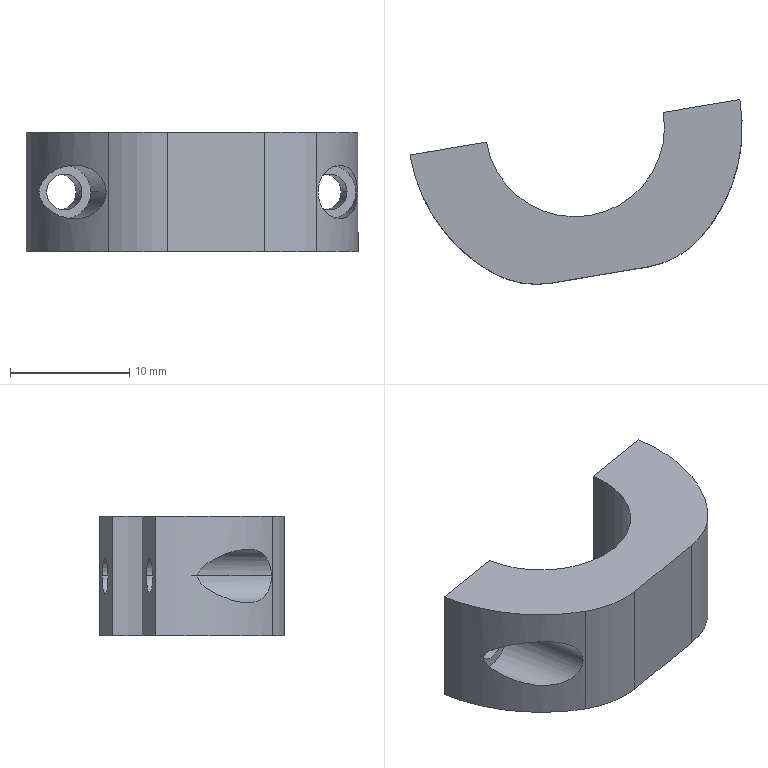Component | SolidWorks | ConnectingRod1-1-1 | 1 solid | 21 faces | box 27.81 x 15.47 x 10 mm | volume 1858 mm3 | cylinder 14 | plane 7 | commonest cylinder face diameters 4.5 x4 3 x4 15 x4 28 x2
build123d program:
from build123d import *

# Parameters (mm, degrees)
BOSS_EXTRUDE1_DEPTH = 20
SKETCH2_R           = 6
CUT_EXTRUDE1_DEPTH  = 12
SKETCH3_R           = 9
CUT_EXTRUDE2_DEPTH  = 74.973
SKETCH4_W           = 60.236
SKETCH4_H           = 18.31
CUT_EXTRUDE3_DEPTH  = 89.724
FILLET1_R           = 30
SCALE1_SCALE        = 0.25


with BuildPart() as part:
    # Sketch1 → Boss-Extrude1 (new, symmetric)
    with BuildSketch(Plane(origin=(0, 0, 0), x_dir=(1, 0, 0), z_dir=(0, 1, 0))):
        with BuildLine():
            Line((-56, 0), (-30, 0))
            ThreePointArc((-30, 0), (0, 30), (30, 0))
            Line((30, 0), (56, 0))
            ThreePointArc((56, 0), (0, 56), (-56, 0))
        make_face()
    extrude(amount=BOSS_EXTRUDE1_DEPTH, both=True)

    # Sketch2 → Cut-Extrude1 (cut)
    with BuildSketch(Plane.XY):
        with Locations((-45, 0)):
            Circle(SKETCH2_R)
        with Locations((45, 0)):
            Circle(SKETCH2_R)
    extrude(amount=-CUT_EXTRUDE1_DEPTH, mode=Mode.SUBTRACT)

    # Sketch3 → Cut-Extrude2 (cut, through all)
    with BuildSketch(Plane.XY.offset(-12)):
        with Locations((-45, 0)):
            Circle(SKETCH3_R)
        with Locations((45, 0)):
            Circle(SKETCH3_R)
    extrude(amount=-CUT_EXTRUDE2_DEPTH, mode=Mode.SUBTRACT)

    # Sketch4 → Cut-Extrude3 (cut, through all)
    with BuildSketch(Plane(origin=(0, 20, 0), x_dir=(1, 0, 0), z_dir=(0, 1, 0))):
        with Locations((0, 59.315)):
            Rectangle(SKETCH4_W, SKETCH4_H)
    extrude(amount=-CUT_EXTRUDE3_DEPTH, mode=Mode.SUBTRACT)

    # Fillet1
    fillet1_edges = [part.edges().sort_by_distance(p)[0] for p in [
        (-24.9, 0, -50.159),
        (24.9, 0, -50.159),
    ]]
    fillet(fillet1_edges, radius=FILLET1_R)


with BuildPart() as part_1:
    # Scale1: scaled about (-0.001703, 6.1763e-05, -27.435)
    add(part.part.scale(SCALE1_SCALE).moved(Location((-0.001278, 0.00004632, -20.576))))


solid = part_1.part

# Placed as in the assembly
solid = solid.moved(Location((39.229, -232.365, 206.462), (-90, -9.535, 0.0002559)))
STEP:
#1=COLOUR_RGB('',0.7922,0.8196,0.9333);
#2=FILL_AREA_STYLE_COLOUR('',#1);
#3=FILL_AREA_STYLE('',(#2));
#4=SURFACE_STYLE_FILL_AREA(#3);
#5=SURFACE_SIDE_STYLE('',(#4));
#6=SURFACE_STYLE_USAGE(.BOTH.,#5);
#7=PRESENTATION_STYLE_ASSIGNMENT((#6));
#8=CARTESIAN_POINT('',(2.098,-10.305,8.128));
#9=VERTEX_POINT('',#8);
#10=CARTESIAN_POINT('',(2.227,-10.003,8.128));
#11=VERTEX_POINT('',#10);
#12=CARTESIAN_POINT('',(2.098,-10.305,8.128));
#13=CARTESIAN_POINT('',(2.098,-10.305,8.133));
#14=CARTESIAN_POINT('',(2.098,-10.304,8.137));
#15=CARTESIAN_POINT('',(2.099,-10.303,8.145));
#16=CARTESIAN_POINT('',(2.1,-10.302,8.149));
#17=CARTESIAN_POINT('',(2.103,-10.299,8.161));
#18=CARTESIAN_POINT('',(2.106,-10.295,8.169));
#19=CARTESIAN_POINT('',(2.113,-10.287,8.182));
#20=CARTESIAN_POINT('',(2.117,-10.282,8.188));
#21=CARTESIAN_POINT('',(2.125,-10.27,8.197));
#22=CARTESIAN_POINT('',(2.129,-10.264,8.201));
#23=CARTESIAN_POINT('',(2.138,-10.251,8.208));
#24=CARTESIAN_POINT('',(2.143,-10.244,8.21));
#25=CARTESIAN_POINT('',(2.152,-10.23,8.214));
#26=CARTESIAN_POINT('',(2.156,-10.223,8.215));
#27=CARTESIAN_POINT('',(2.168,-10.201,8.218));
#28=CARTESIAN_POINT('',(2.176,-10.186,8.217));
#29=CARTESIAN_POINT('',(2.189,-10.155,8.214));
#30=CARTESIAN_POINT('',(2.195,-10.139,8.21));
#31=CARTESIAN_POINT('',(2.206,-10.108,8.202));
#32=CARTESIAN_POINT('',(2.21,-10.093,8.196));
#33=CARTESIAN_POINT('',(2.216,-10.07,8.187));
#34=CARTESIAN_POINT('',(2.218,-10.063,8.184));
#35=CARTESIAN_POINT('',(2.221,-10.048,8.176));
#36=CARTESIAN_POINT('',(2.222,-10.041,8.172));
#37=CARTESIAN_POINT('',(2.224,-10.027,8.163));
#38=CARTESIAN_POINT('',(2.225,-10.02,8.157));
#39=CARTESIAN_POINT('',(2.226,-10.011,8.148));
#40=CARTESIAN_POINT('',(2.226,-10.008,8.145));
#41=CARTESIAN_POINT('',(2.227,-10.004,8.137));
#42=CARTESIAN_POINT('',(2.227,-10.003,8.133));
#43=CARTESIAN_POINT('',(2.227,-10.003,8.128));
#44=B_SPLINE_CURVE_WITH_KNOTS('',3,(#12,#13,#14,#15,#16,#17,#18,#19,#20,#21,#22,#23,#24,#25,#26,#27,#28,#29,#30,#31,#32,#33,#34,#35,#36,#37,#38,#39,#40,#41,#42,#43),.UNSPECIFIED.,.F.,.F.,(4,2,2,2,2,2,2,2,2,2,2,2,2,2,2,4),(0.0104,0.01073,0.01105,0.0117,0.01235,0.013,0.01365,0.0143,0.0156,0.0169,0.0182,0.01885,0.0195,0.02015,0.02047,0.0208),.UNSPECIFIED.);
#45=EDGE_CURVE('',#9,#11,#44,.T.);
#46=ORIENTED_EDGE('',*,*,#45,.F.);
#47=CARTESIAN_POINT('',(2.048,-10.005,8.128));
#48=VERTEX_POINT('',#47);
#49=CARTESIAN_POINT('',(2.119,-10.432,8.128));
#50=DIRECTION('',(-0.1656,0.9862,-0.));
#51=VECTOR('',#50,39.37);
#52=LINE('',#49,#51);
#53=EDGE_CURVE('',#9,#48,#52,.T.);
#54=ORIENTED_EDGE('',*,*,#53,.T.);
#55=CARTESIAN_POINT('',(2.222,-9.976,8.128));
#56=VERTEX_POINT('',#55);
#57=CARTESIAN_POINT('',(2.135,-9.99,8.128));
#58=DIRECTION('',(-0.1656,0.9862,-0.));
#59=DIRECTION('',(0.9862,0.1656,0.));
#60=AXIS2_PLACEMENT_3D('',#57,#58,#59);
#61=CIRCLE('',#60,0.08858);
#62=EDGE_CURVE('',#48,#56,#61,.T.);
#63=ORIENTED_EDGE('',*,*,#62,.T.);
#64=CARTESIAN_POINT('',(2.294,-10.403,8.128));
#65=DIRECTION('',(-0.1656,0.9862,-0.));
#66=VECTOR('',#65,39.37);
#67=LINE('',#64,#66);
#68=EDGE_CURVE('',#11,#56,#67,.T.);
#69=ORIENTED_EDGE('',*,*,#68,.F.);
#70=EDGE_LOOP('',(#46,#54,#63,#69));
#71=FACE_OUTER_BOUND('',#70,.T.);
#72=CARTESIAN_POINT('',(2.207,-10.417,8.128));
#73=DIRECTION('',(-0.1656,0.9862,-0.));
#74=DIRECTION('',(0.9862,0.1656,0.));
#75=AXIS2_PLACEMENT_3D('',#72,#73,#74);
#76=CYLINDRICAL_SURFACE('',#75,0.08858);
#77=ADVANCED_FACE('',(#71),#76,.F.);
#78=CARTESIAN_POINT('',(1.179,-10.179,8.128));
#79=VERTEX_POINT('',#78);
#80=CARTESIAN_POINT('',(1.399,-10.422,8.128));
#81=VERTEX_POINT('',#80);
#82=CARTESIAN_POINT('',(1.179,-10.179,8.128));
#83=CARTESIAN_POINT('',(1.179,-10.179,8.133));
#84=CARTESIAN_POINT('',(1.179,-10.18,8.137));
#85=CARTESIAN_POINT('',(1.181,-10.184,8.145));
#86=CARTESIAN_POINT('',(1.182,-10.186,8.148));
#87=CARTESIAN_POINT('',(1.186,-10.194,8.157));
#88=CARTESIAN_POINT('',(1.189,-10.2,8.163));
#89=CARTESIAN_POINT('',(1.196,-10.213,8.172));
#90=CARTESIAN_POINT('',(1.199,-10.219,8.176));
#91=CARTESIAN_POINT('',(1.207,-10.232,8.184));
#92=CARTESIAN_POINT('',(1.211,-10.239,8.187));
#93=CARTESIAN_POINT('',(1.224,-10.259,8.197));
#94=CARTESIAN_POINT('',(1.233,-10.272,8.202));
#95=CARTESIAN_POINT('',(1.253,-10.298,8.21));
#96=CARTESIAN_POINT('',(1.264,-10.31,8.214));
#97=CARTESIAN_POINT('',(1.281,-10.329,8.216));
#98=CARTESIAN_POINT('',(1.287,-10.335,8.217));
#99=CARTESIAN_POINT('',(1.299,-10.347,8.217));
#100=CARTESIAN_POINT('',(1.305,-10.353,8.217));
#101=CARTESIAN_POINT('',(1.318,-10.364,8.215));
#102=CARTESIAN_POINT('',(1.324,-10.369,8.214));
#103=CARTESIAN_POINT('',(1.337,-10.38,8.21));
#104=CARTESIAN_POINT('',(1.343,-10.385,8.208));
#105=CARTESIAN_POINT('',(1.356,-10.394,8.201));
#106=CARTESIAN_POINT('',(1.362,-10.399,8.197));
#107=CARTESIAN_POINT('',(1.374,-10.406,8.188));
#108=CARTESIAN_POINT('',(1.379,-10.41,8.182));
#109=CARTESIAN_POINT('',(1.386,-10.414,8.172));
#110=CARTESIAN_POINT('',(1.388,-10.416,8.169));
#111=CARTESIAN_POINT('',(1.392,-10.418,8.161));
#112=CARTESIAN_POINT('',(1.394,-10.419,8.158));
#113=CARTESIAN_POINT('',(1.396,-10.421,8.15));
#114=CARTESIAN_POINT('',(1.397,-10.421,8.145));
#115=CARTESIAN_POINT('',(1.399,-10.422,8.137));
#116=CARTESIAN_POINT('',(1.399,-10.422,8.133));
#117=CARTESIAN_POINT('',(1.399,-10.422,8.128));
#118=B_SPLINE_CURVE_WITH_KNOTS('',3,(#82,#83,#84,#85,#86,#87,#88,#89,#90,#91,#92,#93,#94,#95,#96,#97,#98,#99,#100,#101,#102,#103,#104,#105,#106,#107,#108,#109,#110,#111,#112,#113,#114,#115,#116,#117),.UNSPECIFIED.,.F.,.F.,(4,2,2,2,2,2,2,2,2,2,2,2,2,2,2,2,2,4),(0.01035,0.01068,0.011,0.01165,0.01229,0.01294,0.01424,0.01553,0.01618,0.01682,0.01747,0.01812,0.01876,0.01941,0.01973,0.02006,0.02038,0.0207),.UNSPECIFIED.);
#119=EDGE_CURVE('',#79,#81,#118,.T.);
#120=ORIENTED_EDGE('',*,*,#119,.F.);
#121=CARTESIAN_POINT('',(1.174,-10.152,8.128));
#122=VERTEX_POINT('',#121);
#123=CARTESIAN_POINT('',(1.246,-10.579,8.128));
#124=DIRECTION('',(-0.1656,0.9862,-0.));
#125=VECTOR('',#124,39.37);
#126=LINE('',#123,#125);
#127=EDGE_CURVE('',#79,#122,#126,.T.);
#128=ORIENTED_EDGE('',*,*,#127,.T.);
#129=CARTESIAN_POINT('',(1.349,-10.122,8.128));
#130=VERTEX_POINT('',#129);
#131=CARTESIAN_POINT('',(1.261,-10.137,8.128));
#132=DIRECTION('',(-0.1656,0.9862,-0.));
#133=DIRECTION('',(0.9862,0.1656,0.));
#134=AXIS2_PLACEMENT_3D('',#131,#132,#133);
#135=CIRCLE('',#134,0.08858);
#136=EDGE_CURVE('',#122,#130,#135,.T.);
#137=ORIENTED_EDGE('',*,*,#136,.T.);
#138=CARTESIAN_POINT('',(1.42,-10.549,8.128));
#139=DIRECTION('',(-0.1656,0.9862,-0.));
#140=VECTOR('',#139,39.37);
#141=LINE('',#138,#140);
#142=EDGE_CURVE('',#81,#130,#141,.T.);
#143=ORIENTED_EDGE('',*,*,#142,.F.);
#144=EDGE_LOOP('',(#120,#128,#137,#143));
#145=FACE_OUTER_BOUND('',#144,.T.);
#146=CARTESIAN_POINT('',(1.333,-10.564,8.128));
#147=DIRECTION('',(-0.1656,0.9862,-0.));
#148=DIRECTION('',(0.9862,0.1656,0.));
#149=AXIS2_PLACEMENT_3D('',#146,#147,#148);
#150=CYLINDRICAL_SURFACE('',#149,0.08858);
#151=ADVANCED_FACE('',(#145),#150,.F.);
#152=CARTESIAN_POINT('',(2.193,-9.98,8.128));
#153=VERTEX_POINT('',#152);
#154=CARTESIAN_POINT('',(2.077,-10.,8.128));
#155=VERTEX_POINT('',#154);
#156=CARTESIAN_POINT('',(2.135,-9.99,8.128));
#157=DIRECTION('',(0.1656,-0.9862,0.));
#158=DIRECTION('',(0.9862,0.1656,0.));
#159=AXIS2_PLACEMENT_3D('',#156,#157,#158);
#160=CIRCLE('',#159,0.05906);
#161=EDGE_CURVE('',#153,#155,#160,.T.);
#162=ORIENTED_EDGE('',*,*,#161,.T.);
#163=CARTESIAN_POINT('',(2.057,-9.884,8.128));
#164=VERTEX_POINT('',#163);
#165=CARTESIAN_POINT('',(2.077,-10.,8.128));
#166=DIRECTION('',(-0.1656,0.9862,-0.));
#167=VECTOR('',#166,39.37);
#168=LINE('',#165,#167);
#169=EDGE_CURVE('',#155,#164,#168,.T.);
#170=ORIENTED_EDGE('',*,*,#169,.T.);
#171=CARTESIAN_POINT('',(2.174,-9.864,8.128));
#172=VERTEX_POINT('',#171);
#173=CARTESIAN_POINT('',(2.115,-9.874,8.128));
#174=DIRECTION('',(-0.1656,0.9862,-0.));
#175=DIRECTION('',(0.9862,0.1656,0.));
#176=AXIS2_PLACEMENT_3D('',#173,#174,#175);
#177=CIRCLE('',#176,0.05906);
#178=EDGE_CURVE('',#164,#172,#177,.T.);
#179=ORIENTED_EDGE('',*,*,#178,.T.);
#180=CARTESIAN_POINT('',(2.193,-9.98,8.128));
#181=DIRECTION('',(-0.1656,0.9862,-0.));
#182=VECTOR('',#181,39.37);
#183=LINE('',#180,#182);
#184=EDGE_CURVE('',#153,#172,#183,.T.);
#185=ORIENTED_EDGE('',*,*,#184,.F.);
#186=EDGE_LOOP('',(#162,#170,#179,#185));
#187=FACE_OUTER_BOUND('',#186,.T.);
#188=CARTESIAN_POINT('',(2.135,-9.99,8.128));
#189=DIRECTION('',(-0.1656,0.9862,-0.));
#190=DIRECTION('',(0.9862,0.1656,0.));
#191=AXIS2_PLACEMENT_3D('',#188,#189,#190);
#192=CYLINDRICAL_SURFACE('',#191,0.05906);
#193=ADVANCED_FACE('',(#187),#192,.F.);
#194=CARTESIAN_POINT('',(1.32,-10.127,8.128));
#195=VERTEX_POINT('',#194);
#196=CARTESIAN_POINT('',(1.203,-10.147,8.128));
#197=VERTEX_POINT('',#196);
#198=CARTESIAN_POINT('',(1.261,-10.137,8.128));
#199=DIRECTION('',(0.1656,-0.9862,0.));
#200=DIRECTION('',(0.9862,0.1656,0.));
#201=AXIS2_PLACEMENT_3D('',#198,#199,#200);
#202=CIRCLE('',#201,0.05906);
#203=EDGE_CURVE('',#195,#197,#202,.T.);
#204=ORIENTED_EDGE('',*,*,#203,.T.);
#205=CARTESIAN_POINT('',(1.184,-10.03,8.128));
#206=VERTEX_POINT('',#205);
#207=CARTESIAN_POINT('',(1.203,-10.147,8.128));
#208=DIRECTION('',(-0.1656,0.9862,-0.));
#209=VECTOR('',#208,39.37);
#210=LINE('',#207,#209);
#211=EDGE_CURVE('',#197,#206,#210,.T.);
#212=ORIENTED_EDGE('',*,*,#211,.T.);
#213=CARTESIAN_POINT('',(1.3,-10.011,8.128));
#214=VERTEX_POINT('',#213);
#215=CARTESIAN_POINT('',(1.242,-10.02,8.128));
#216=DIRECTION('',(-0.1656,0.9862,-0.));
#217=DIRECTION('',(0.9862,0.1656,0.));
#218=AXIS2_PLACEMENT_3D('',#215,#216,#217);
#219=CIRCLE('',#218,0.05906);
#220=EDGE_CURVE('',#206,#214,#219,.T.);
#221=ORIENTED_EDGE('',*,*,#220,.T.);
#222=CARTESIAN_POINT('',(1.32,-10.127,8.128));
#223=DIRECTION('',(-0.1656,0.9862,-0.));
#224=VECTOR('',#223,39.37);
#225=LINE('',#222,#224);
#226=EDGE_CURVE('',#195,#214,#225,.T.);
#227=ORIENTED_EDGE('',*,*,#226,.F.);
#228=EDGE_LOOP('',(#204,#212,#221,#227));
#229=FACE_OUTER_BOUND('',#228,.T.);
#230=CARTESIAN_POINT('',(1.261,-10.137,8.128));
#231=DIRECTION('',(-0.1656,0.9862,-0.));
#232=DIRECTION('',(0.9862,0.1656,0.));
#233=AXIS2_PLACEMENT_3D('',#230,#231,#232);
#234=CYLINDRICAL_SURFACE('',#233,0.05906);
#235=ADVANCED_FACE('',(#229),#234,.F.);
#236=CARTESIAN_POINT('',(1.727,-10.238,7.932));
#237=VERTEX_POINT('',#236);
#238=CARTESIAN_POINT('',(1.97,-9.898,7.932));
#239=VERTEX_POINT('',#238);
#240=CARTESIAN_POINT('',(1.679,-9.947,7.932));
#241=DIRECTION('',(-0.,0.,1.));
#242=DIRECTION('',(-0.1656,0.9862,0.));
#243=AXIS2_PLACEMENT_3D('',#240,#241,#242);
#244=CIRCLE('',#243,0.2953);
#245=EDGE_CURVE('',#237,#239,#244,.T.);
#246=ORIENTED_EDGE('',*,*,#245,.F.);
#247=CARTESIAN_POINT('',(1.727,-10.238,8.325));
#248=VERTEX_POINT('',#247);
#249=CARTESIAN_POINT('',(1.727,-10.238,7.932));
#250=DIRECTION('',(-0.,0.,1.));
#251=VECTOR('',#250,39.37);
#252=LINE('',#249,#251);
#253=EDGE_CURVE('',#237,#248,#252,.T.);
#254=ORIENTED_EDGE('',*,*,#253,.T.);
#255=CARTESIAN_POINT('',(1.97,-9.898,8.325));
#256=VERTEX_POINT('',#255);
#257=CARTESIAN_POINT('',(1.679,-9.947,8.325));
#258=DIRECTION('',(-0.,0.,1.));
#259=DIRECTION('',(-0.1656,0.9862,0.));
#260=AXIS2_PLACEMENT_3D('',#257,#258,#259);
#261=CIRCLE('',#260,0.2953);
#262=EDGE_CURVE('',#248,#256,#261,.T.);
#263=ORIENTED_EDGE('',*,*,#262,.T.);
#264=CARTESIAN_POINT('',(1.97,-9.898,7.932));
#265=DIRECTION('',(-0.,0.,1.));
#266=VECTOR('',#265,39.37);
#267=LINE('',#264,#266);
#268=EDGE_CURVE('',#239,#256,#267,.T.);
#269=ORIENTED_EDGE('',*,*,#268,.F.);
#270=EDGE_LOOP('',(#246,#254,#263,#269));
#271=FACE_OUTER_BOUND('',#270,.T.);
#272=CARTESIAN_POINT('',(1.679,-9.947,7.932));
#273=DIRECTION('',(-0.,0.,1.));
#274=DIRECTION('',(0.1656,-0.9862,0.));
#275=AXIS2_PLACEMENT_3D('',#272,#273,#274);
#276=CYLINDRICAL_SURFACE('',#275,0.2953);
#277=ADVANCED_FACE('',(#271),#276,.F.);
#278=CARTESIAN_POINT('',(1.399,-10.422,8.128));
#279=CARTESIAN_POINT('',(1.399,-10.422,8.12));
#280=CARTESIAN_POINT('',(1.398,-10.421,8.111));
#281=CARTESIAN_POINT('',(1.392,-10.418,8.095));
#282=CARTESIAN_POINT('',(1.389,-10.416,8.088));
#283=CARTESIAN_POINT('',(1.379,-10.41,8.075));
#284=CARTESIAN_POINT('',(1.374,-10.406,8.069));
#285=CARTESIAN_POINT('',(1.362,-10.398,8.06));
#286=CARTESIAN_POINT('',(1.356,-10.394,8.056));
#287=CARTESIAN_POINT('',(1.343,-10.385,8.049));
#288=CARTESIAN_POINT('',(1.337,-10.38,8.047));
#289=CARTESIAN_POINT('',(1.324,-10.369,8.043));
#290=CARTESIAN_POINT('',(1.318,-10.364,8.042));
#291=CARTESIAN_POINT('',(1.305,-10.353,8.04));
#292=CARTESIAN_POINT('',(1.299,-10.347,8.04));
#293=CARTESIAN_POINT('',(1.287,-10.335,8.04));
#294=CARTESIAN_POINT('',(1.281,-10.329,8.041));
#295=CARTESIAN_POINT('',(1.264,-10.31,8.043));
#296=CARTESIAN_POINT('',(1.253,-10.298,8.047));
#297=CARTESIAN_POINT('',(1.233,-10.272,8.055));
#298=CARTESIAN_POINT('',(1.224,-10.259,8.06));
#299=CARTESIAN_POINT('',(1.211,-10.239,8.07));
#300=CARTESIAN_POINT('',(1.207,-10.232,8.073));
#301=CARTESIAN_POINT('',(1.199,-10.219,8.081));
#302=CARTESIAN_POINT('',(1.196,-10.213,8.085));
#303=CARTESIAN_POINT('',(1.189,-10.2,8.094));
#304=CARTESIAN_POINT('',(1.186,-10.194,8.1));
#305=CARTESIAN_POINT('',(1.182,-10.186,8.109));
#306=CARTESIAN_POINT('',(1.181,-10.184,8.112));
#307=CARTESIAN_POINT('',(1.179,-10.18,8.12));
#308=CARTESIAN_POINT('',(1.179,-10.179,8.124));
#309=CARTESIAN_POINT('',(1.179,-10.179,8.128));
#310=B_SPLINE_CURVE_WITH_KNOTS('',3,(#278,#279,#280,#281,#282,#283,#284,#285,#286,#287,#288,#289,#290,#291,#292,#293,#294,#295,#296,#297,#298,#299,#300,#301,#302,#303,#304,#305,#306,#307,#308,#309),.UNSPECIFIED.,.F.,.F.,(4,2,2,2,2,2,2,2,2,2,2,2,2,2,2,4),(0.,0.0006471,0.001294,0.001941,0.002589,0.003236,0.003883,0.00453,0.005177,0.006471,0.007766,0.008413,0.00906,0.009707,0.01003,0.01035),.UNSPECIFIED.);
#311=EDGE_CURVE('',#81,#79,#310,.T.);
#312=ORIENTED_EDGE('',*,*,#311,.T.);
#313=ORIENTED_EDGE('',*,*,#119,.T.);
#314=EDGE_LOOP('',(#312,#313));
#315=FACE_BOUND('',#314,.T.);
#316=CARTESIAN_POINT('',(1.406,-10.426,7.932));
#317=VERTEX_POINT('',#316);
#318=CARTESIAN_POINT('',(1.135,-10.038,7.932));
#319=VERTEX_POINT('',#318);
#320=CARTESIAN_POINT('',(1.679,-9.947,7.932));
#321=DIRECTION('',(0.,-0.,-1.));
#322=DIRECTION('',(-0.1656,0.9862,0.));
#323=AXIS2_PLACEMENT_3D('',#320,#321,#322);
#324=CIRCLE('',#323,0.5512);
#325=EDGE_CURVE('',#317,#319,#324,.T.);
#326=ORIENTED_EDGE('',*,*,#325,.F.);
#327=CARTESIAN_POINT('',(1.406,-10.426,8.325));
#328=VERTEX_POINT('',#327);
#329=CARTESIAN_POINT('',(1.406,-10.426,7.932));
#330=DIRECTION('',(-0.,0.,1.));
#331=VECTOR('',#330,39.37);
#332=LINE('',#329,#331);
#333=EDGE_CURVE('',#317,#328,#332,.T.);
#334=ORIENTED_EDGE('',*,*,#333,.T.);
#335=CARTESIAN_POINT('',(1.135,-10.038,8.325));
#336=VERTEX_POINT('',#335);
#337=CARTESIAN_POINT('',(1.679,-9.947,8.325));
#338=DIRECTION('',(0.,-0.,-1.));
#339=DIRECTION('',(-0.1656,0.9862,0.));
#340=AXIS2_PLACEMENT_3D('',#337,#338,#339);
#341=CIRCLE('',#340,0.5512);
#342=EDGE_CURVE('',#328,#336,#341,.T.);
#343=ORIENTED_EDGE('',*,*,#342,.T.);
#344=CARTESIAN_POINT('',(1.135,-10.038,7.932));
#345=DIRECTION('',(-0.,0.,1.));
#346=VECTOR('',#345,39.37);
#347=LINE('',#344,#346);
#348=EDGE_CURVE('',#319,#336,#347,.T.);
#349=ORIENTED_EDGE('',*,*,#348,.F.);
#350=EDGE_LOOP('',(#326,#334,#343,#349));
#351=FACE_OUTER_BOUND('',#350,.T.);
#352=CARTESIAN_POINT('',(1.679,-9.947,7.932));
#353=DIRECTION('',(-0.,0.,1.));
#354=DIRECTION('',(0.1656,-0.9862,0.));
#355=AXIS2_PLACEMENT_3D('',#352,#353,#354);
#356=CYLINDRICAL_SURFACE('',#355,0.5512);
#357=ADVANCED_FACE('',(#315,#351),#356,.T.);
#358=ORIENTED_EDGE('',*,*,#253,.F.);
#359=CARTESIAN_POINT('',(1.387,-9.996,7.932));
#360=VERTEX_POINT('',#359);
#361=CARTESIAN_POINT('',(1.679,-9.947,7.932));
#362=DIRECTION('',(-0.,0.,1.));
#363=DIRECTION('',(-0.1656,0.9862,0.));
#364=AXIS2_PLACEMENT_3D('',#361,#362,#363);
#365=CIRCLE('',#364,0.2953);
#366=EDGE_CURVE('',#360,#237,#365,.T.);
#367=ORIENTED_EDGE('',*,*,#366,.F.);
#368=CARTESIAN_POINT('',(1.387,-9.996,8.325));
#369=VERTEX_POINT('',#368);
#370=CARTESIAN_POINT('',(1.387,-9.996,7.932));
#371=DIRECTION('',(-0.,0.,1.));
#372=VECTOR('',#371,39.37);
#373=LINE('',#370,#372);
#374=EDGE_CURVE('',#360,#369,#373,.T.);
#375=ORIENTED_EDGE('',*,*,#374,.T.);
#376=CARTESIAN_POINT('',(1.679,-9.947,8.325));
#377=DIRECTION('',(-0.,0.,1.));
#378=DIRECTION('',(-0.1656,0.9862,0.));
#379=AXIS2_PLACEMENT_3D('',#376,#377,#378);
#380=CIRCLE('',#379,0.2953);
#381=EDGE_CURVE('',#369,#248,#380,.T.);
#382=ORIENTED_EDGE('',*,*,#381,.T.);
#383=EDGE_LOOP('',(#358,#367,#375,#382));
#384=FACE_OUTER_BOUND('',#383,.T.);
#385=CARTESIAN_POINT('',(1.679,-9.947,7.932));
#386=DIRECTION('',(-0.,0.,1.));
#387=DIRECTION('',(0.1656,-0.9862,0.));
#388=AXIS2_PLACEMENT_3D('',#385,#386,#387);
#389=CYLINDRICAL_SURFACE('',#388,0.2953);
#390=ADVANCED_FACE('',(#384),#389,.F.);
#391=CARTESIAN_POINT('',(2.115,-9.874,8.128));
#392=DIRECTION('',(-0.1656,0.9862,-0.));
#393=DIRECTION('',(0.9862,0.1656,0.));
#394=AXIS2_PLACEMENT_3D('',#391,#392,#393);
#395=CIRCLE('',#394,0.05906);
#396=EDGE_CURVE('',#172,#164,#395,.T.);
#397=ORIENTED_EDGE('',*,*,#396,.F.);
#398=ORIENTED_EDGE('',*,*,#178,.F.);
#399=EDGE_LOOP('',(#397,#398));
#400=FACE_BOUND('',#399,.T.);
#401=CARTESIAN_POINT('',(2.222,-9.856,8.325));
#402=VERTEX_POINT('',#401);
#403=CARTESIAN_POINT('',(1.97,-9.898,8.325));
#404=DIRECTION('',(0.9862,0.1656,0.));
#405=VECTOR('',#404,39.37);
#406=LINE('',#403,#405);
#407=EDGE_CURVE('',#256,#402,#406,.T.);
#408=ORIENTED_EDGE('',*,*,#407,.T.);
#409=CARTESIAN_POINT('',(2.222,-9.856,7.932));
#410=VERTEX_POINT('',#409);
#411=CARTESIAN_POINT('',(2.222,-9.856,7.932));
#412=DIRECTION('',(-0.,0.,1.));
#413=VECTOR('',#412,39.37);
#414=LINE('',#411,#413);
#415=EDGE_CURVE('',#410,#402,#414,.T.);
#416=ORIENTED_EDGE('',*,*,#415,.F.);
#417=CARTESIAN_POINT('',(1.97,-9.898,7.932));
#418=DIRECTION('',(0.9862,0.1656,0.));
#419=VECTOR('',#418,39.37);
#420=LINE('',#417,#419);
#421=EDGE_CURVE('',#239,#410,#420,.T.);
#422=ORIENTED_EDGE('',*,*,#421,.F.);
#423=ORIENTED_EDGE('',*,*,#268,.T.);
#424=EDGE_LOOP('',(#408,#416,#422,#423));
#425=FACE_OUTER_BOUND('',#424,.T.);
#426=CARTESIAN_POINT('',(1.97,-9.898,7.932));
#427=DIRECTION('',(0.1656,-0.9862,0.));
#428=DIRECTION('',(-0.9862,-0.1656,-0.));
#429=AXIS2_PLACEMENT_3D('',#426,#427,#428);
#430=PLANE('',#429);
#431=ADVANCED_FACE('',(#400,#425),#430,.F.);
#432=CARTESIAN_POINT('',(2.227,-10.003,8.128));
#433=CARTESIAN_POINT('',(2.227,-10.003,8.124));
#434=CARTESIAN_POINT('',(2.227,-10.004,8.12));
#435=CARTESIAN_POINT('',(2.226,-10.008,8.112));
#436=CARTESIAN_POINT('',(2.226,-10.011,8.109));
#437=CARTESIAN_POINT('',(2.225,-10.02,8.099));
#438=CARTESIAN_POINT('',(2.224,-10.026,8.094));
#439=CARTESIAN_POINT('',(2.222,-10.04,8.085));
#440=CARTESIAN_POINT('',(2.221,-10.048,8.081));
#441=CARTESIAN_POINT('',(2.218,-10.063,8.073));
#442=CARTESIAN_POINT('',(2.216,-10.07,8.07));
#443=CARTESIAN_POINT('',(2.21,-10.093,8.06));
#444=CARTESIAN_POINT('',(2.206,-10.108,8.055));
#445=CARTESIAN_POINT('',(2.195,-10.14,8.047));
#446=CARTESIAN_POINT('',(2.189,-10.155,8.043));
#447=CARTESIAN_POINT('',(2.179,-10.178,8.041));
#448=CARTESIAN_POINT('',(2.176,-10.186,8.04));
#449=CARTESIAN_POINT('',(2.168,-10.201,8.04));
#450=CARTESIAN_POINT('',(2.164,-10.208,8.04));
#451=CARTESIAN_POINT('',(2.156,-10.223,8.042));
#452=CARTESIAN_POINT('',(2.152,-10.23,8.043));
#453=CARTESIAN_POINT('',(2.143,-10.244,8.047));
#454=CARTESIAN_POINT('',(2.138,-10.251,8.049));
#455=CARTESIAN_POINT('',(2.129,-10.264,8.056));
#456=CARTESIAN_POINT('',(2.125,-10.27,8.06));
#457=CARTESIAN_POINT('',(2.117,-10.282,8.069));
#458=CARTESIAN_POINT('',(2.113,-10.287,8.075));
#459=CARTESIAN_POINT('',(2.108,-10.293,8.085));
#460=CARTESIAN_POINT('',(2.106,-10.295,8.088));
#461=CARTESIAN_POINT('',(2.103,-10.299,8.096));
#462=CARTESIAN_POINT('',(2.102,-10.3,8.099));
#463=CARTESIAN_POINT('',(2.1,-10.302,8.107));
#464=CARTESIAN_POINT('',(2.099,-10.303,8.112));
#465=CARTESIAN_POINT('',(2.098,-10.304,8.12));
#466=CARTESIAN_POINT('',(2.098,-10.305,8.124));
#467=CARTESIAN_POINT('',(2.098,-10.305,8.128));
#468=B_SPLINE_CURVE_WITH_KNOTS('',3,(#432,#433,#434,#435,#436,#437,#438,#439,#440,#441,#442,#443,#444,#445,#446,#447,#448,#449,#450,#451,#452,#453,#454,#455,#456,#457,#458,#459,#460,#461,#462,#463,#464,#465,#466,#467),.UNSPECIFIED.,.F.,.F.,(4,2,2,2,2,2,2,2,2,2,2,2,2,2,2,2,2,4),(0.,0.0003251,0.0006502,0.0013,0.001951,0.002601,0.003901,0.005202,0.005852,0.006502,0.007153,0.007803,0.008453,0.009103,0.009429,0.009754,0.01008,0.0104),.UNSPECIFIED.);
#469=EDGE_CURVE('',#11,#9,#468,.T.);
#470=ORIENTED_EDGE('',*,*,#469,.T.);
#471=ORIENTED_EDGE('',*,*,#45,.T.);
#472=EDGE_LOOP('',(#470,#471));
#473=FACE_BOUND('',#472,.T.);
#474=CARTESIAN_POINT('',(2.093,-10.311,8.325));
#475=VERTEX_POINT('',#474);
#476=CARTESIAN_POINT('',(1.679,-9.947,8.325));
#477=DIRECTION('',(0.,-0.,-1.));
#478=DIRECTION('',(-0.1656,0.9862,0.));
#479=AXIS2_PLACEMENT_3D('',#476,#477,#478);
#480=CIRCLE('',#479,0.5512);
#481=EDGE_CURVE('',#402,#475,#480,.T.);
#482=ORIENTED_EDGE('',*,*,#481,.T.);
#483=CARTESIAN_POINT('',(2.093,-10.311,7.932));
#484=VERTEX_POINT('',#483);
#485=CARTESIAN_POINT('',(2.093,-10.311,7.932));
#486=DIRECTION('',(0.,-0.,-1.));
#487=VECTOR('',#486,39.37);
#488=LINE('',#485,#487);
#489=EDGE_CURVE('',#475,#484,#488,.T.);
#490=ORIENTED_EDGE('',*,*,#489,.T.);
#491=CARTESIAN_POINT('',(1.679,-9.947,7.932));
#492=DIRECTION('',(0.,-0.,-1.));
#493=DIRECTION('',(-0.1656,0.9862,0.));
#494=AXIS2_PLACEMENT_3D('',#491,#492,#493);
#495=CIRCLE('',#494,0.5512);
#496=EDGE_CURVE('',#410,#484,#495,.T.);
#497=ORIENTED_EDGE('',*,*,#496,.F.);
#498=ORIENTED_EDGE('',*,*,#415,.T.);
#499=EDGE_LOOP('',(#482,#490,#497,#498));
#500=FACE_OUTER_BOUND('',#499,.T.);
#501=CARTESIAN_POINT('',(1.679,-9.947,7.932));
#502=DIRECTION('',(-0.,0.,1.));
#503=DIRECTION('',(0.1656,-0.9862,0.));
#504=AXIS2_PLACEMENT_3D('',#501,#502,#503);
#505=CYLINDRICAL_SURFACE('',#504,0.5512);
#506=ADVANCED_FACE('',(#473,#500),#505,.T.);
#507=CARTESIAN_POINT('',(1.242,-10.02,8.128));
#508=DIRECTION('',(-0.1656,0.9862,-0.));
#509=DIRECTION('',(0.9862,0.1656,0.));
#510=AXIS2_PLACEMENT_3D('',#507,#508,#509);
#511=CIRCLE('',#510,0.05906);
#512=EDGE_CURVE('',#214,#206,#511,.T.);
#513=ORIENTED_EDGE('',*,*,#512,.F.);
#514=ORIENTED_EDGE('',*,*,#220,.F.);
#515=EDGE_LOOP('',(#513,#514));
#516=FACE_BOUND('',#515,.T.);
#517=CARTESIAN_POINT('',(1.135,-10.038,8.325));
#518=DIRECTION('',(0.9862,0.1656,0.));
#519=VECTOR('',#518,39.37);
#520=LINE('',#517,#519);
#521=EDGE_CURVE('',#336,#369,#520,.T.);
#522=ORIENTED_EDGE('',*,*,#521,.T.);
#523=ORIENTED_EDGE('',*,*,#374,.F.);
#524=CARTESIAN_POINT('',(1.135,-10.038,7.932));
#525=DIRECTION('',(0.9862,0.1656,0.));
#526=VECTOR('',#525,39.37);
#527=LINE('',#524,#526);
#528=EDGE_CURVE('',#319,#360,#527,.T.);
#529=ORIENTED_EDGE('',*,*,#528,.F.);
#530=ORIENTED_EDGE('',*,*,#348,.T.);
#531=EDGE_LOOP('',(#522,#523,#529,#530));
#532=FACE_OUTER_BOUND('',#531,.T.);
#533=CARTESIAN_POINT('',(1.135,-10.038,7.932));
#534=DIRECTION('',(0.1656,-0.9862,0.));
#535=DIRECTION('',(-0.9862,-0.1656,-0.));
#536=AXIS2_PLACEMENT_3D('',#533,#534,#535);
#537=PLANE('',#536);
#538=ADVANCED_FACE('',(#516,#532),#537,.F.);
#539=CARTESIAN_POINT('',(1.601,-10.461,7.932));
#540=VERTEX_POINT('',#539);
#541=CARTESIAN_POINT('',(1.92,-10.407,7.932));
#542=VERTEX_POINT('',#541);
#543=CARTESIAN_POINT('',(1.468,-10.483,7.932));
#544=DIRECTION('',(0.9862,0.1656,0.));
#545=VECTOR('',#544,39.37);
#546=LINE('',#543,#545);
#547=EDGE_CURVE('',#540,#542,#546,.T.);
#548=ORIENTED_EDGE('',*,*,#547,.F.);
#549=CARTESIAN_POINT('',(1.552,-10.17,7.932));
#550=DIRECTION('',(0.,-0.,-1.));
#551=DIRECTION('',(-0.1656,0.9862,0.));
#552=AXIS2_PLACEMENT_3D('',#549,#550,#551);
#553=CIRCLE('',#552,0.2953);
#554=EDGE_CURVE('',#540,#317,#553,.T.);
#555=ORIENTED_EDGE('',*,*,#554,.T.);
#556=ORIENTED_EDGE('',*,*,#325,.T.);
#557=ORIENTED_EDGE('',*,*,#528,.T.);
#558=ORIENTED_EDGE('',*,*,#366,.T.);
#559=ORIENTED_EDGE('',*,*,#245,.T.);
#560=ORIENTED_EDGE('',*,*,#421,.T.);
#561=ORIENTED_EDGE('',*,*,#496,.T.);
#562=CARTESIAN_POINT('',(1.871,-10.116,7.932));
#563=DIRECTION('',(0.,-0.,-1.));
#564=DIRECTION('',(-0.1656,0.9862,0.));
#565=AXIS2_PLACEMENT_3D('',#562,#563,#564);
#566=CIRCLE('',#565,0.2953);
#567=EDGE_CURVE('',#484,#542,#566,.T.);
#568=ORIENTED_EDGE('',*,*,#567,.T.);
#569=EDGE_LOOP('',(#548,#555,#556,#557,#558,#559,#560,#561,#568));
#570=FACE_OUTER_BOUND('',#569,.T.);
#571=CARTESIAN_POINT('',(1.679,-9.947,7.932));
#572=DIRECTION('',(0.,-0.,-1.));
#573=DIRECTION('',(-0.1656,0.9862,-0.));
#574=AXIS2_PLACEMENT_3D('',#571,#572,#573);
#575=PLANE('',#574);
#576=ADVANCED_FACE('',(#570),#575,.T.);
#577=ORIENTED_EDGE('',*,*,#342,.F.);
#578=CARTESIAN_POINT('',(1.601,-10.461,8.325));
#579=VERTEX_POINT('',#578);
#580=CARTESIAN_POINT('',(1.552,-10.17,8.325));
#581=DIRECTION('',(-0.,0.,1.));
#582=DIRECTION('',(-0.1656,0.9862,0.));
#583=AXIS2_PLACEMENT_3D('',#580,#581,#582);
#584=CIRCLE('',#583,0.2953);
#585=EDGE_CURVE('',#328,#579,#584,.T.);
#586=ORIENTED_EDGE('',*,*,#585,.T.);
#587=CARTESIAN_POINT('',(1.92,-10.407,8.325));
#588=VERTEX_POINT('',#587);
#589=CARTESIAN_POINT('',(1.76,-10.434,8.325));
#590=DIRECTION('',(0.9862,0.1656,0.));
#591=VECTOR('',#590,39.37);
#592=LINE('',#589,#591);
#593=EDGE_CURVE('',#579,#588,#592,.T.);
#594=ORIENTED_EDGE('',*,*,#593,.T.);
#595=CARTESIAN_POINT('',(1.871,-10.116,8.325));
#596=DIRECTION('',(-0.,0.,1.));
#597=DIRECTION('',(-0.1656,0.9862,0.));
#598=AXIS2_PLACEMENT_3D('',#595,#596,#597);
#599=CIRCLE('',#598,0.2953);
#600=EDGE_CURVE('',#588,#475,#599,.T.);
#601=ORIENTED_EDGE('',*,*,#600,.T.);
#602=ORIENTED_EDGE('',*,*,#481,.F.);
#603=ORIENTED_EDGE('',*,*,#407,.F.);
#604=ORIENTED_EDGE('',*,*,#262,.F.);
#605=ORIENTED_EDGE('',*,*,#381,.F.);
#606=ORIENTED_EDGE('',*,*,#521,.F.);
#607=EDGE_LOOP('',(#577,#586,#594,#601,#602,#603,#604,#605,#606));
#608=FACE_OUTER_BOUND('',#607,.T.);
#609=CARTESIAN_POINT('',(1.679,-9.947,8.325));
#610=DIRECTION('',(0.,-0.,-1.));
#611=DIRECTION('',(-0.1656,0.9862,-0.));
#612=AXIS2_PLACEMENT_3D('',#609,#610,#611);
#613=PLANE('',#612);
#614=ADVANCED_FACE('',(#608),#613,.F.);
#615=ORIENTED_EDGE('',*,*,#211,.F.);
#616=CARTESIAN_POINT('',(1.261,-10.137,8.128));
#617=DIRECTION('',(0.1656,-0.9862,0.));
#618=DIRECTION('',(0.9862,0.1656,0.));
#619=AXIS2_PLACEMENT_3D('',#616,#617,#618);
#620=CIRCLE('',#619,0.05906);
#621=EDGE_CURVE('',#197,#195,#620,.T.);
#622=ORIENTED_EDGE('',*,*,#621,.T.);
#623=ORIENTED_EDGE('',*,*,#226,.T.);
#624=ORIENTED_EDGE('',*,*,#512,.T.);
#625=EDGE_LOOP('',(#615,#622,#623,#624));
#626=FACE_OUTER_BOUND('',#625,.T.);
#627=CARTESIAN_POINT('',(1.261,-10.137,8.128));
#628=DIRECTION('',(-0.1656,0.9862,-0.));
#629=DIRECTION('',(0.9862,0.1656,0.));
#630=AXIS2_PLACEMENT_3D('',#627,#628,#629);
#631=CYLINDRICAL_SURFACE('',#630,0.05906);
#632=ADVANCED_FACE('',(#626),#631,.F.);
#633=ORIENTED_EDGE('',*,*,#169,.F.);
#634=CARTESIAN_POINT('',(2.135,-9.99,8.128));
#635=DIRECTION('',(0.1656,-0.9862,0.));
#636=DIRECTION('',(0.9862,0.1656,0.));
#637=AXIS2_PLACEMENT_3D('',#634,#635,#636);
#638=CIRCLE('',#637,0.05906);
#639=EDGE_CURVE('',#155,#153,#638,.T.);
#640=ORIENTED_EDGE('',*,*,#639,.T.);
#641=ORIENTED_EDGE('',*,*,#184,.T.);
#642=ORIENTED_EDGE('',*,*,#396,.T.);
#643=EDGE_LOOP('',(#633,#640,#641,#642));
#644=FACE_OUTER_BOUND('',#643,.T.);
#645=CARTESIAN_POINT('',(2.135,-9.99,8.128));
#646=DIRECTION('',(-0.1656,0.9862,-0.));
#647=DIRECTION('',(0.9862,0.1656,0.));
#648=AXIS2_PLACEMENT_3D('',#645,#646,#647);
#649=CYLINDRICAL_SURFACE('',#648,0.05906);
#650=ADVANCED_FACE('',(#644),#649,.F.);
#651=ORIENTED_EDGE('',*,*,#127,.F.);
#652=ORIENTED_EDGE('',*,*,#311,.F.);
#653=ORIENTED_EDGE('',*,*,#142,.T.);
#654=CARTESIAN_POINT('',(1.261,-10.137,8.128));
#655=DIRECTION('',(-0.1656,0.9862,-0.));
#656=DIRECTION('',(0.9862,0.1656,0.));
#657=AXIS2_PLACEMENT_3D('',#654,#655,#656);
#658=CIRCLE('',#657,0.08858);
#659=EDGE_CURVE('',#130,#122,#658,.T.);
#660=ORIENTED_EDGE('',*,*,#659,.T.);
#661=EDGE_LOOP('',(#651,#652,#653,#660));
#662=FACE_OUTER_BOUND('',#661,.T.);
#663=CARTESIAN_POINT('',(1.333,-10.564,8.128));
#664=DIRECTION('',(-0.1656,0.9862,-0.));
#665=DIRECTION('',(0.9862,0.1656,0.));
#666=AXIS2_PLACEMENT_3D('',#663,#664,#665);
#667=CYLINDRICAL_SURFACE('',#666,0.08858);
#668=ADVANCED_FACE('',(#662),#667,.F.);
#669=ORIENTED_EDGE('',*,*,#659,.F.);
#670=ORIENTED_EDGE('',*,*,#136,.F.);
#671=EDGE_LOOP('',(#669,#670));
#672=FACE_OUTER_BOUND('',#671,.T.);
#673=ORIENTED_EDGE('',*,*,#203,.F.);
#674=ORIENTED_EDGE('',*,*,#621,.F.);
#675=EDGE_LOOP('',(#673,#674));
#676=FACE_BOUND('',#675,.T.);
#677=CARTESIAN_POINT('',(1.261,-10.137,8.128));
#678=DIRECTION('',(-0.1656,0.9862,-0.));
#679=DIRECTION('',(0.9862,0.1656,0.));
#680=AXIS2_PLACEMENT_3D('',#677,#678,#679);
#681=PLANE('',#680);
#682=ADVANCED_FACE('',(#672,#676),#681,.F.);
#683=ORIENTED_EDGE('',*,*,#53,.F.);
#684=ORIENTED_EDGE('',*,*,#469,.F.);
#685=ORIENTED_EDGE('',*,*,#68,.T.);
#686=CARTESIAN_POINT('',(2.135,-9.99,8.128));
#687=DIRECTION('',(-0.1656,0.9862,-0.));
#688=DIRECTION('',(0.9862,0.1656,0.));
#689=AXIS2_PLACEMENT_3D('',#686,#687,#688);
#690=CIRCLE('',#689,0.08858);
#691=EDGE_CURVE('',#56,#48,#690,.T.);
#692=ORIENTED_EDGE('',*,*,#691,.T.);
#693=EDGE_LOOP('',(#683,#684,#685,#692));
#694=FACE_OUTER_BOUND('',#693,.T.);
#695=CARTESIAN_POINT('',(2.207,-10.417,8.128));
#696=DIRECTION('',(-0.1656,0.9862,-0.));
#697=DIRECTION('',(0.9862,0.1656,0.));
#698=AXIS2_PLACEMENT_3D('',#695,#696,#697);
#699=CYLINDRICAL_SURFACE('',#698,0.08858);
#700=ADVANCED_FACE('',(#694),#699,.F.);
#701=ORIENTED_EDGE('',*,*,#691,.F.);
#702=ORIENTED_EDGE('',*,*,#62,.F.);
#703=EDGE_LOOP('',(#701,#702));
#704=FACE_OUTER_BOUND('',#703,.T.);
#705=ORIENTED_EDGE('',*,*,#161,.F.);
#706=ORIENTED_EDGE('',*,*,#639,.F.);
#707=EDGE_LOOP('',(#705,#706));
#708=FACE_BOUND('',#707,.T.);
#709=CARTESIAN_POINT('',(2.135,-9.99,8.128));
#710=DIRECTION('',(-0.1656,0.9862,-0.));
#711=DIRECTION('',(0.9862,0.1656,0.));
#712=AXIS2_PLACEMENT_3D('',#709,#710,#711);
#713=PLANE('',#712);
#714=ADVANCED_FACE('',(#704,#708),#713,.F.);
#715=ORIENTED_EDGE('',*,*,#593,.F.);
#716=CARTESIAN_POINT('',(1.601,-10.461,8.325));
#717=DIRECTION('',(0.,-0.,-1.));
#718=VECTOR('',#717,39.37);
#719=LINE('',#716,#718);
#720=EDGE_CURVE('',#579,#540,#719,.T.);
#721=ORIENTED_EDGE('',*,*,#720,.T.);
#722=ORIENTED_EDGE('',*,*,#547,.T.);
#723=CARTESIAN_POINT('',(1.92,-10.407,8.325));
#724=DIRECTION('',(-0.,0.,1.));
#725=VECTOR('',#724,39.37);
#726=LINE('',#723,#725);
#727=EDGE_CURVE('',#542,#588,#726,.T.);
#728=ORIENTED_EDGE('',*,*,#727,.T.);
#729=EDGE_LOOP('',(#715,#721,#722,#728));
#730=FACE_OUTER_BOUND('',#729,.T.);
#731=CARTESIAN_POINT('',(1.468,-10.483,8.325));
#732=DIRECTION('',(-0.1656,0.9862,-0.));
#733=DIRECTION('',(0.9862,0.1656,0.));
#734=AXIS2_PLACEMENT_3D('',#731,#732,#733);
#735=PLANE('',#734);
#736=ADVANCED_FACE('',(#730),#735,.F.);
#737=ORIENTED_EDGE('',*,*,#554,.F.);
#738=ORIENTED_EDGE('',*,*,#720,.F.);
#739=ORIENTED_EDGE('',*,*,#585,.F.);
#740=ORIENTED_EDGE('',*,*,#333,.F.);
#741=EDGE_LOOP('',(#737,#738,#739,#740));
#742=FACE_OUTER_BOUND('',#741,.T.);
#743=CARTESIAN_POINT('',(1.552,-10.17,7.932));
#744=DIRECTION('',(-0.,0.,1.));
#745=DIRECTION('',(0.1656,-0.9862,0.));
#746=AXIS2_PLACEMENT_3D('',#743,#744,#745);
#747=CYLINDRICAL_SURFACE('',#746,0.2953);
#748=ADVANCED_FACE('',(#742),#747,.T.);
#749=ORIENTED_EDGE('',*,*,#600,.F.);
#750=ORIENTED_EDGE('',*,*,#727,.F.);
#751=ORIENTED_EDGE('',*,*,#567,.F.);
#752=ORIENTED_EDGE('',*,*,#489,.F.);
#753=EDGE_LOOP('',(#749,#750,#751,#752));
#754=FACE_OUTER_BOUND('',#753,.T.);
#755=CARTESIAN_POINT('',(1.871,-10.116,7.932));
#756=DIRECTION('',(-0.,0.,1.));
#757=DIRECTION('',(0.1656,-0.9862,0.));
#758=AXIS2_PLACEMENT_3D('',#755,#756,#757);
#759=CYLINDRICAL_SURFACE('',#758,0.2953);
#760=ADVANCED_FACE('',(#754),#759,.T.);
#761=CLOSED_SHELL('',(#77,#151,#193,#235,#277,#357,#390,#431,#506,#538,#576,#614,#632,#650,#668,#682,#700,#714,#736,#748,#760));
#762=MANIFOLD_SOLID_BREP('',#761);
#763=STYLED_ITEM('',(#7),#762);
#764=(LENGTH_UNIT()NAMED_UNIT(*)SI_UNIT($,.METRE.));
#765=LENGTH_MEASURE_WITH_UNIT(LENGTH_MEASURE(0.0254),#764);
#766=DIMENSIONAL_EXPONENTS(1.,0.,0.,0.,0.,0.,0.);
#767=(CONVERSION_BASED_UNIT('',#765)LENGTH_UNIT()NAMED_UNIT(#766));
#768=UNCERTAINTY_MEASURE_WITH_UNIT(LENGTH_MEASURE(0.00001),#767,'','');
#769=(NAMED_UNIT(*)PLANE_ANGLE_UNIT()SI_UNIT($,.RADIAN.));
#770=(NAMED_UNIT(*)SI_UNIT($,.STERADIAN.)SOLID_ANGLE_UNIT());
#771=(GEOMETRIC_REPRESENTATION_CONTEXT(3)GLOBAL_UNCERTAINTY_ASSIGNED_CONTEXT((#768))GLOBAL_UNIT_ASSIGNED_CONTEXT((#767,#769,#770))REPRESENTATION_CONTEXT('',''));
#772=MECHANICAL_DESIGN_GEOMETRIC_PRESENTATION_REPRESENTATION('',(#763),#771);
#773=CARTESIAN_POINT('',(0.,0.,0.));
#774=DIRECTION('',(0.,0.,1.));
#775=DIRECTION('',(1.,0.,0.));
#776=AXIS2_PLACEMENT_3D('',#773,#774,#775);
#777=(LENGTH_UNIT()NAMED_UNIT(*)SI_UNIT($,.METRE.));
#778=LENGTH_MEASURE_WITH_UNIT(LENGTH_MEASURE(0.0254),#777);
#779=DIMENSIONAL_EXPONENTS(1.,0.,0.,0.,0.,0.,0.);
#780=(CONVERSION_BASED_UNIT('',#778)LENGTH_UNIT()NAMED_UNIT(#779));
#781=UNCERTAINTY_MEASURE_WITH_UNIT(LENGTH_MEASURE(0.00001),#780,'','');
#782=(NAMED_UNIT(*)PLANE_ANGLE_UNIT()SI_UNIT($,.RADIAN.));
#783=(NAMED_UNIT(*)SI_UNIT($,.STERADIAN.)SOLID_ANGLE_UNIT());
#784=(GEOMETRIC_REPRESENTATION_CONTEXT(3)GLOBAL_UNCERTAINTY_ASSIGNED_CONTEXT((#781))GLOBAL_UNIT_ASSIGNED_CONTEXT((#780,#782,#783))REPRESENTATION_CONTEXT('',''));
#785=ADVANCED_BREP_SHAPE_REPRESENTATION('',(#762,#776),#784);
#786=PRESENTATION_LAYER_ASSIGNMENT('','',(#763));